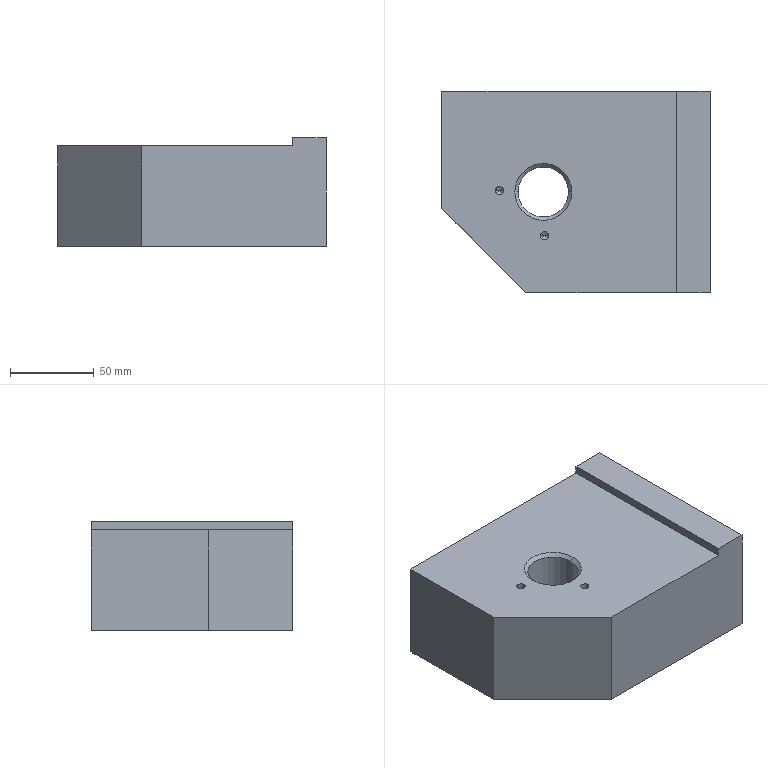Component | SolidWorks | JF21-80.1-1-3(_)-1-SOLID57-1 | 1 solid | 23 faces | box 160 x 120 x 65 mm | volume 1045468 mm3 | plane 9 | cone 8 | cylinder 6 | commonest cylinder face diameters 5 x4 30 x2
STEP:
#1=CARTESIAN_POINT('',(11.241,-3.767,39.961));
#2=VERTEX_POINT('',#1);
#3=CARTESIAN_POINT('',(12.422,-3.767,39.961));
#4=VERTEX_POINT('',#3);
#5=CARTESIAN_POINT('',(11.832,-3.767,39.961));
#6=DIRECTION('',(0.,0.,1.));
#7=DIRECTION('',(1.,0.,0.));
#8=AXIS2_PLACEMENT_3D('',#5,#6,#7);
#9=CIRCLE('',#8,0.5906);
#10=EDGE_CURVE('',#2,#4,#9,.T.);
#11=ORIENTED_EDGE('',*,*,#10,.F.);
#12=CARTESIAN_POINT('',(11.162,-3.767,40.039));
#13=VERTEX_POINT('',#12);
#14=CARTESIAN_POINT('',(11.241,-3.767,39.961));
#15=DIRECTION('',(-0.7071,0.,0.7071));
#16=VECTOR('',#15,39.37);
#17=LINE('',#14,#16);
#18=EDGE_CURVE('',#2,#13,#17,.T.);
#19=ORIENTED_EDGE('',*,*,#18,.T.);
#20=CARTESIAN_POINT('',(12.501,-3.767,40.039));
#21=VERTEX_POINT('',#20);
#22=CARTESIAN_POINT('',(11.832,-3.767,40.039));
#23=DIRECTION('',(0.,0.,-1.));
#24=DIRECTION('',(1.,0.,0.));
#25=AXIS2_PLACEMENT_3D('',#22,#23,#24);
#26=CIRCLE('',#25,0.6693);
#27=EDGE_CURVE('',#21,#13,#26,.T.);
#28=ORIENTED_EDGE('',*,*,#27,.F.);
#29=CARTESIAN_POINT('',(12.422,-3.767,39.961));
#30=DIRECTION('',(0.7071,0.,0.7071));
#31=VECTOR('',#30,39.37);
#32=LINE('',#29,#31);
#33=EDGE_CURVE('',#4,#21,#32,.T.);
#34=ORIENTED_EDGE('',*,*,#33,.F.);
#35=EDGE_LOOP('',(#11,#19,#28,#34));
#36=FACE_OUTER_BOUND('',#35,.T.);
#37=CARTESIAN_POINT('',(11.832,-3.767,39.961));
#38=DIRECTION('',(0.,0.,1.));
#39=DIRECTION('',(-1.,0.,0.));
#40=AXIS2_PLACEMENT_3D('',#37,#38,#39);
#41=CONICAL_SURFACE('',#40,0.5906,0.7854);
#42=ADVANCED_FACE('',(#36),#41,.F.);
#43=CARTESIAN_POINT('',(12.422,-3.767,37.756));
#44=VERTEX_POINT('',#43);
#45=CARTESIAN_POINT('',(11.241,-3.767,37.756));
#46=VERTEX_POINT('',#45);
#47=CARTESIAN_POINT('',(11.832,-3.767,37.756));
#48=DIRECTION('',(0.,0.,-1.));
#49=DIRECTION('',(-1.,0.,0.));
#50=AXIS2_PLACEMENT_3D('',#47,#48,#49);
#51=CIRCLE('',#50,0.5906);
#52=EDGE_CURVE('',#44,#46,#51,.T.);
#53=ORIENTED_EDGE('',*,*,#52,.F.);
#54=CARTESIAN_POINT('',(12.501,-3.767,37.677));
#55=VERTEX_POINT('',#54);
#56=CARTESIAN_POINT('',(12.501,-3.767,37.677));
#57=DIRECTION('',(-0.7071,-0.,0.7071));
#58=VECTOR('',#57,39.37);
#59=LINE('',#56,#58);
#60=EDGE_CURVE('',#55,#44,#59,.T.);
#61=ORIENTED_EDGE('',*,*,#60,.F.);
#62=CARTESIAN_POINT('',(11.162,-3.767,37.677));
#63=VERTEX_POINT('',#62);
#64=CARTESIAN_POINT('',(11.832,-3.767,37.677));
#65=DIRECTION('',(0.,0.,1.));
#66=DIRECTION('',(-1.,0.,0.));
#67=AXIS2_PLACEMENT_3D('',#64,#65,#66);
#68=CIRCLE('',#67,0.6693);
#69=EDGE_CURVE('',#63,#55,#68,.T.);
#70=ORIENTED_EDGE('',*,*,#69,.F.);
#71=CARTESIAN_POINT('',(11.162,-3.767,37.677));
#72=DIRECTION('',(0.7071,0.,0.7071));
#73=VECTOR('',#72,39.37);
#74=LINE('',#71,#73);
#75=EDGE_CURVE('',#63,#46,#74,.T.);
#76=ORIENTED_EDGE('',*,*,#75,.T.);
#77=EDGE_LOOP('',(#53,#61,#70,#76));
#78=FACE_OUTER_BOUND('',#77,.T.);
#79=CARTESIAN_POINT('',(11.832,-3.767,37.677));
#80=DIRECTION('',(0.,0.,-1.));
#81=DIRECTION('',(1.,0.,0.));
#82=AXIS2_PLACEMENT_3D('',#79,#80,#81);
#83=CONICAL_SURFACE('',#82,0.6693,0.7854);
#84=ADVANCED_FACE('',(#78),#83,.F.);
#85=CARTESIAN_POINT('',(10.703,-3.739,39.331));
#86=VERTEX_POINT('',#85);
#87=CARTESIAN_POINT('',(10.9,-3.739,39.331));
#88=VERTEX_POINT('',#87);
#89=CARTESIAN_POINT('',(10.801,-3.739,39.331));
#90=DIRECTION('',(0.,0.,1.));
#91=DIRECTION('',(1.,0.,0.));
#92=AXIS2_PLACEMENT_3D('',#89,#90,#91);
#93=CIRCLE('',#92,0.09843);
#94=EDGE_CURVE('',#86,#88,#93,.T.);
#95=ORIENTED_EDGE('',*,*,#94,.F.);
#96=CARTESIAN_POINT('',(10.703,-3.739,40.039));
#97=VERTEX_POINT('',#96);
#98=CARTESIAN_POINT('',(10.703,-3.739,40.039));
#99=DIRECTION('',(0.,0.,1.));
#100=VECTOR('',#99,39.37);
#101=LINE('',#98,#100);
#102=EDGE_CURVE('',#86,#97,#101,.T.);
#103=ORIENTED_EDGE('',*,*,#102,.T.);
#104=CARTESIAN_POINT('',(10.9,-3.739,40.039));
#105=VERTEX_POINT('',#104);
#106=CARTESIAN_POINT('',(10.801,-3.739,40.039));
#107=DIRECTION('',(0.,0.,1.));
#108=DIRECTION('',(1.,0.,0.));
#109=AXIS2_PLACEMENT_3D('',#106,#107,#108);
#110=CIRCLE('',#109,0.09843);
#111=EDGE_CURVE('',#97,#105,#110,.T.);
#112=ORIENTED_EDGE('',*,*,#111,.T.);
#113=CARTESIAN_POINT('',(10.9,-3.739,40.039));
#114=DIRECTION('',(0.,0.,1.));
#115=VECTOR('',#114,39.37);
#116=LINE('',#113,#115);
#117=EDGE_CURVE('',#88,#105,#116,.T.);
#118=ORIENTED_EDGE('',*,*,#117,.F.);
#119=EDGE_LOOP('',(#95,#103,#112,#118));
#120=FACE_OUTER_BOUND('',#119,.T.);
#121=CARTESIAN_POINT('',(10.801,-3.739,40.039));
#122=DIRECTION('',(0.,0.,1.));
#123=DIRECTION('',(-1.,0.,0.));
#124=AXIS2_PLACEMENT_3D('',#121,#122,#123);
#125=CYLINDRICAL_SURFACE('',#124,0.09843);
#126=ADVANCED_FACE('',(#120),#125,.F.);
#127=CARTESIAN_POINT('',(10.801,-3.739,39.272));
#128=VERTEX_POINT('',#127);
#129=CARTESIAN_POINT('',(10.9,-3.739,39.331));
#130=DIRECTION('',(0.8572,0.,0.515));
#131=VECTOR('',#130,39.37);
#132=LINE('',#129,#131);
#133=EDGE_CURVE('',#128,#88,#132,.T.);
#134=ORIENTED_EDGE('',*,*,#133,.F.);
#135=CARTESIAN_POINT('',(10.703,-3.739,39.331));
#136=DIRECTION('',(-0.8572,0.,0.515));
#137=VECTOR('',#136,39.37);
#138=LINE('',#135,#137);
#139=EDGE_CURVE('',#128,#86,#138,.T.);
#140=ORIENTED_EDGE('',*,*,#139,.T.);
#141=ORIENTED_EDGE('',*,*,#94,.T.);
#142=EDGE_LOOP('',(#134,#140,#141));
#143=FACE_OUTER_BOUND('',#142,.T.);
#144=CARTESIAN_POINT('',(10.801,-3.739,39.331));
#145=DIRECTION('',(0.,0.,1.));
#146=DIRECTION('',(-1.,0.,0.));
#147=AXIS2_PLACEMENT_3D('',#144,#145,#146);
#148=CONICAL_SURFACE('',#147,0.09843,1.03);
#149=ADVANCED_FACE('',(#143),#148,.F.);
#150=CARTESIAN_POINT('',(11.761,-4.797,39.331));
#151=VERTEX_POINT('',#150);
#152=CARTESIAN_POINT('',(11.958,-4.797,39.331));
#153=VERTEX_POINT('',#152);
#154=CARTESIAN_POINT('',(11.859,-4.797,39.331));
#155=DIRECTION('',(0.,0.,1.));
#156=DIRECTION('',(1.,0.,0.));
#157=AXIS2_PLACEMENT_3D('',#154,#155,#156);
#158=CIRCLE('',#157,0.09843);
#159=EDGE_CURVE('',#151,#153,#158,.T.);
#160=ORIENTED_EDGE('',*,*,#159,.F.);
#161=CARTESIAN_POINT('',(11.761,-4.797,40.039));
#162=VERTEX_POINT('',#161);
#163=CARTESIAN_POINT('',(11.761,-4.797,40.039));
#164=DIRECTION('',(0.,0.,1.));
#165=VECTOR('',#164,39.37);
#166=LINE('',#163,#165);
#167=EDGE_CURVE('',#151,#162,#166,.T.);
#168=ORIENTED_EDGE('',*,*,#167,.T.);
#169=CARTESIAN_POINT('',(11.958,-4.797,40.039));
#170=VERTEX_POINT('',#169);
#171=CARTESIAN_POINT('',(11.859,-4.797,40.039));
#172=DIRECTION('',(0.,0.,1.));
#173=DIRECTION('',(1.,0.,0.));
#174=AXIS2_PLACEMENT_3D('',#171,#172,#173);
#175=CIRCLE('',#174,0.09843);
#176=EDGE_CURVE('',#162,#170,#175,.T.);
#177=ORIENTED_EDGE('',*,*,#176,.T.);
#178=CARTESIAN_POINT('',(11.958,-4.797,40.039));
#179=DIRECTION('',(0.,0.,1.));
#180=VECTOR('',#179,39.37);
#181=LINE('',#178,#180);
#182=EDGE_CURVE('',#153,#170,#181,.T.);
#183=ORIENTED_EDGE('',*,*,#182,.F.);
#184=EDGE_LOOP('',(#160,#168,#177,#183));
#185=FACE_OUTER_BOUND('',#184,.T.);
#186=CARTESIAN_POINT('',(11.859,-4.797,40.039));
#187=DIRECTION('',(0.,0.,1.));
#188=DIRECTION('',(-1.,0.,0.));
#189=AXIS2_PLACEMENT_3D('',#186,#187,#188);
#190=CYLINDRICAL_SURFACE('',#189,0.09843);
#191=ADVANCED_FACE('',(#185),#190,.F.);
#192=CARTESIAN_POINT('',(11.859,-4.797,39.272));
#193=VERTEX_POINT('',#192);
#194=CARTESIAN_POINT('',(11.958,-4.797,39.331));
#195=DIRECTION('',(0.8572,0.,0.515));
#196=VECTOR('',#195,39.37);
#197=LINE('',#194,#196);
#198=EDGE_CURVE('',#193,#153,#197,.T.);
#199=ORIENTED_EDGE('',*,*,#198,.F.);
#200=CARTESIAN_POINT('',(11.761,-4.797,39.331));
#201=DIRECTION('',(-0.8572,0.,0.515));
#202=VECTOR('',#201,39.37);
#203=LINE('',#200,#202);
#204=EDGE_CURVE('',#193,#151,#203,.T.);
#205=ORIENTED_EDGE('',*,*,#204,.T.);
#206=ORIENTED_EDGE('',*,*,#159,.T.);
#207=EDGE_LOOP('',(#199,#205,#206));
#208=FACE_OUTER_BOUND('',#207,.T.);
#209=CARTESIAN_POINT('',(11.859,-4.797,39.331));
#210=DIRECTION('',(0.,0.,1.));
#211=DIRECTION('',(-1.,0.,0.));
#212=AXIS2_PLACEMENT_3D('',#209,#210,#211);
#213=CONICAL_SURFACE('',#212,0.09843,1.03);
#214=ADVANCED_FACE('',(#208),#213,.F.);
#215=ORIENTED_EDGE('',*,*,#10,.T.);
#216=CARTESIAN_POINT('',(12.422,-3.767,40.236));
#217=DIRECTION('',(0.,0.,1.));
#218=VECTOR('',#217,39.37);
#219=LINE('',#216,#218);
#220=EDGE_CURVE('',#44,#4,#219,.T.);
#221=ORIENTED_EDGE('',*,*,#220,.F.);
#222=ORIENTED_EDGE('',*,*,#52,.T.);
#223=CARTESIAN_POINT('',(11.241,-3.767,40.236));
#224=DIRECTION('',(0.,0.,1.));
#225=VECTOR('',#224,39.37);
#226=LINE('',#223,#225);
#227=EDGE_CURVE('',#46,#2,#226,.T.);
#228=ORIENTED_EDGE('',*,*,#227,.T.);
#229=EDGE_LOOP('',(#215,#221,#222,#228));
#230=FACE_OUTER_BOUND('',#229,.T.);
#231=CARTESIAN_POINT('',(11.832,-3.767,40.236));
#232=DIRECTION('',(0.,0.,-1.));
#233=DIRECTION('',(1.,0.,0.));
#234=AXIS2_PLACEMENT_3D('',#231,#232,#233);
#235=CYLINDRICAL_SURFACE('',#234,0.5906);
#236=ADVANCED_FACE('',(#230),#235,.F.);
#237=CARTESIAN_POINT('',(9.449,-1.404,40.039));
#238=VERTEX_POINT('',#237);
#239=CARTESIAN_POINT('',(9.449,-4.16,40.039));
#240=VERTEX_POINT('',#239);
#241=CARTESIAN_POINT('',(9.449,-1.404,40.039));
#242=DIRECTION('',(0.,-1.,0.));
#243=VECTOR('',#242,39.37);
#244=LINE('',#241,#243);
#245=EDGE_CURVE('',#238,#240,#244,.T.);
#246=ORIENTED_EDGE('',*,*,#245,.F.);
#247=CARTESIAN_POINT('',(9.449,-1.404,37.677));
#248=VERTEX_POINT('',#247);
#249=CARTESIAN_POINT('',(9.449,-1.404,40.236));
#250=DIRECTION('',(0.,0.,-1.));
#251=VECTOR('',#250,39.37);
#252=LINE('',#249,#251);
#253=EDGE_CURVE('',#238,#248,#252,.T.);
#254=ORIENTED_EDGE('',*,*,#253,.T.);
#255=CARTESIAN_POINT('',(9.449,-4.16,37.677));
#256=VERTEX_POINT('',#255);
#257=CARTESIAN_POINT('',(9.449,-1.404,37.677));
#258=DIRECTION('',(0.,-1.,0.));
#259=VECTOR('',#258,39.37);
#260=LINE('',#257,#259);
#261=EDGE_CURVE('',#248,#256,#260,.T.);
#262=ORIENTED_EDGE('',*,*,#261,.T.);
#263=CARTESIAN_POINT('',(9.449,-4.16,40.236));
#264=DIRECTION('',(0.,0.,-1.));
#265=VECTOR('',#264,39.37);
#266=LINE('',#263,#265);
#267=EDGE_CURVE('',#240,#256,#266,.T.);
#268=ORIENTED_EDGE('',*,*,#267,.F.);
#269=EDGE_LOOP('',(#246,#254,#262,#268));
#270=FACE_OUTER_BOUND('',#269,.T.);
#271=CARTESIAN_POINT('',(9.449,-1.404,40.236));
#272=DIRECTION('',(1.,0.,0.));
#273=DIRECTION('',(0.,0.,1.));
#274=AXIS2_PLACEMENT_3D('',#271,#272,#273);
#275=PLANE('',#274);
#276=ADVANCED_FACE('',(#270),#275,.F.);
#277=CARTESIAN_POINT('',(11.417,-6.129,40.039));
#278=VERTEX_POINT('',#277);
#279=CARTESIAN_POINT('',(9.449,-4.16,40.039));
#280=DIRECTION('',(0.7071,-0.7071,0.));
#281=VECTOR('',#280,39.37);
#282=LINE('',#279,#281);
#283=EDGE_CURVE('',#240,#278,#282,.T.);
#284=ORIENTED_EDGE('',*,*,#283,.F.);
#285=ORIENTED_EDGE('',*,*,#267,.T.);
#286=CARTESIAN_POINT('',(11.417,-6.129,37.677));
#287=VERTEX_POINT('',#286);
#288=CARTESIAN_POINT('',(9.449,-4.16,37.677));
#289=DIRECTION('',(0.7071,-0.7071,0.));
#290=VECTOR('',#289,39.37);
#291=LINE('',#288,#290);
#292=EDGE_CURVE('',#256,#287,#291,.T.);
#293=ORIENTED_EDGE('',*,*,#292,.T.);
#294=CARTESIAN_POINT('',(11.417,-6.129,40.236));
#295=DIRECTION('',(0.,0.,-1.));
#296=VECTOR('',#295,39.37);
#297=LINE('',#294,#296);
#298=EDGE_CURVE('',#278,#287,#297,.T.);
#299=ORIENTED_EDGE('',*,*,#298,.F.);
#300=EDGE_LOOP('',(#284,#285,#293,#299));
#301=FACE_OUTER_BOUND('',#300,.T.);
#302=CARTESIAN_POINT('',(9.449,-4.16,40.236));
#303=DIRECTION('',(0.7071,0.7071,0.));
#304=DIRECTION('',(0.7071,-0.7071,0.));
#305=AXIS2_PLACEMENT_3D('',#302,#303,#304);
#306=PLANE('',#305);
#307=ADVANCED_FACE('',(#301),#306,.F.);
#308=ORIENTED_EDGE('',*,*,#220,.T.);
#309=CARTESIAN_POINT('',(11.832,-3.767,39.961));
#310=DIRECTION('',(0.,0.,1.));
#311=DIRECTION('',(1.,0.,0.));
#312=AXIS2_PLACEMENT_3D('',#309,#310,#311);
#313=CIRCLE('',#312,0.5906);
#314=EDGE_CURVE('',#4,#2,#313,.T.);
#315=ORIENTED_EDGE('',*,*,#314,.T.);
#316=ORIENTED_EDGE('',*,*,#227,.F.);
#317=CARTESIAN_POINT('',(11.832,-3.767,37.756));
#318=DIRECTION('',(0.,0.,-1.));
#319=DIRECTION('',(-1.,0.,0.));
#320=AXIS2_PLACEMENT_3D('',#317,#318,#319);
#321=CIRCLE('',#320,0.5906);
#322=EDGE_CURVE('',#46,#44,#321,.T.);
#323=ORIENTED_EDGE('',*,*,#322,.T.);
#324=EDGE_LOOP('',(#308,#315,#316,#323));
#325=FACE_OUTER_BOUND('',#324,.T.);
#326=CARTESIAN_POINT('',(11.832,-3.767,40.236));
#327=DIRECTION('',(0.,0.,-1.));
#328=DIRECTION('',(1.,0.,0.));
#329=AXIS2_PLACEMENT_3D('',#326,#327,#328);
#330=CYLINDRICAL_SURFACE('',#329,0.5906);
#331=ADVANCED_FACE('',(#325),#330,.F.);
#332=CARTESIAN_POINT('',(15.748,-1.404,40.236));
#333=VERTEX_POINT('',#332);
#334=CARTESIAN_POINT('',(14.961,-1.404,40.236));
#335=VERTEX_POINT('',#334);
#336=CARTESIAN_POINT('',(15.748,-1.404,40.236));
#337=DIRECTION('',(-1.,-0.,0.));
#338=VECTOR('',#337,39.37);
#339=LINE('',#336,#338);
#340=EDGE_CURVE('',#333,#335,#339,.T.);
#341=ORIENTED_EDGE('',*,*,#340,.T.);
#342=CARTESIAN_POINT('',(14.961,-6.129,40.236));
#343=VERTEX_POINT('',#342);
#344=CARTESIAN_POINT('',(14.961,-1.404,40.236));
#345=DIRECTION('',(0.,1.,0.));
#346=VECTOR('',#345,39.37);
#347=LINE('',#344,#346);
#348=EDGE_CURVE('',#343,#335,#347,.T.);
#349=ORIENTED_EDGE('',*,*,#348,.F.);
#350=CARTESIAN_POINT('',(15.748,-6.129,40.236));
#351=VERTEX_POINT('',#350);
#352=CARTESIAN_POINT('',(15.748,-6.129,40.236));
#353=DIRECTION('',(1.,0.,0.));
#354=VECTOR('',#353,39.37);
#355=LINE('',#352,#354);
#356=EDGE_CURVE('',#343,#351,#355,.T.);
#357=ORIENTED_EDGE('',*,*,#356,.T.);
#358=CARTESIAN_POINT('',(15.748,-1.404,40.236));
#359=DIRECTION('',(0.,1.,0.));
#360=VECTOR('',#359,39.37);
#361=LINE('',#358,#360);
#362=EDGE_CURVE('',#351,#333,#361,.T.);
#363=ORIENTED_EDGE('',*,*,#362,.T.);
#364=EDGE_LOOP('',(#341,#349,#357,#363));
#365=FACE_OUTER_BOUND('',#364,.T.);
#366=CARTESIAN_POINT('',(15.748,-6.129,40.236));
#367=DIRECTION('',(0.,0.,-1.));
#368=DIRECTION('',(1.,0.,0.));
#369=AXIS2_PLACEMENT_3D('',#366,#367,#368);
#370=PLANE('',#369);
#371=ADVANCED_FACE('',(#365),#370,.F.);
#372=ORIENTED_EDGE('',*,*,#69,.T.);
#373=CARTESIAN_POINT('',(11.832,-3.767,37.677));
#374=DIRECTION('',(0.,0.,1.));
#375=DIRECTION('',(-1.,0.,0.));
#376=AXIS2_PLACEMENT_3D('',#373,#374,#375);
#377=CIRCLE('',#376,0.6693);
#378=EDGE_CURVE('',#55,#63,#377,.T.);
#379=ORIENTED_EDGE('',*,*,#378,.T.);
#380=EDGE_LOOP('',(#372,#379));
#381=FACE_BOUND('',#380,.T.);
#382=CARTESIAN_POINT('',(15.748,-6.129,37.677));
#383=VERTEX_POINT('',#382);
#384=CARTESIAN_POINT('',(15.748,-1.404,37.677));
#385=VERTEX_POINT('',#384);
#386=CARTESIAN_POINT('',(15.748,-1.404,37.677));
#387=DIRECTION('',(0.,1.,0.));
#388=VECTOR('',#387,39.37);
#389=LINE('',#386,#388);
#390=EDGE_CURVE('',#383,#385,#389,.T.);
#391=ORIENTED_EDGE('',*,*,#390,.F.);
#392=CARTESIAN_POINT('',(15.748,-6.129,37.677));
#393=DIRECTION('',(1.,0.,0.));
#394=VECTOR('',#393,39.37);
#395=LINE('',#392,#394);
#396=EDGE_CURVE('',#287,#383,#395,.T.);
#397=ORIENTED_EDGE('',*,*,#396,.F.);
#398=ORIENTED_EDGE('',*,*,#292,.F.);
#399=ORIENTED_EDGE('',*,*,#261,.F.);
#400=CARTESIAN_POINT('',(15.748,-1.404,37.677));
#401=DIRECTION('',(-1.,-0.,0.));
#402=VECTOR('',#401,39.37);
#403=LINE('',#400,#402);
#404=EDGE_CURVE('',#385,#248,#403,.T.);
#405=ORIENTED_EDGE('',*,*,#404,.F.);
#406=EDGE_LOOP('',(#391,#397,#398,#399,#405));
#407=FACE_OUTER_BOUND('',#406,.T.);
#408=CARTESIAN_POINT('',(15.748,-6.129,37.677));
#409=DIRECTION('',(0.,0.,-1.));
#410=DIRECTION('',(1.,0.,0.));
#411=AXIS2_PLACEMENT_3D('',#408,#409,#410);
#412=PLANE('',#411);
#413=ADVANCED_FACE('',(#381,#407),#412,.T.);
#414=ORIENTED_EDGE('',*,*,#390,.T.);
#415=CARTESIAN_POINT('',(15.748,-1.404,40.236));
#416=DIRECTION('',(0.,0.,-1.));
#417=VECTOR('',#416,39.37);
#418=LINE('',#415,#417);
#419=EDGE_CURVE('',#333,#385,#418,.T.);
#420=ORIENTED_EDGE('',*,*,#419,.F.);
#421=ORIENTED_EDGE('',*,*,#362,.F.);
#422=CARTESIAN_POINT('',(15.748,-6.129,40.236));
#423=DIRECTION('',(0.,0.,-1.));
#424=VECTOR('',#423,39.37);
#425=LINE('',#422,#424);
#426=EDGE_CURVE('',#351,#383,#425,.T.);
#427=ORIENTED_EDGE('',*,*,#426,.T.);
#428=EDGE_LOOP('',(#414,#420,#421,#427));
#429=FACE_OUTER_BOUND('',#428,.T.);
#430=CARTESIAN_POINT('',(15.748,-1.404,40.236));
#431=DIRECTION('',(-1.,0.,0.));
#432=DIRECTION('',(0.,0.,-1.));
#433=AXIS2_PLACEMENT_3D('',#430,#431,#432);
#434=PLANE('',#433);
#435=ADVANCED_FACE('',(#429),#434,.F.);
#436=CARTESIAN_POINT('',(14.961,-1.404,40.039));
#437=VERTEX_POINT('',#436);
#438=CARTESIAN_POINT('',(14.961,-1.404,40.039));
#439=DIRECTION('',(-1.,-0.,0.));
#440=VECTOR('',#439,39.37);
#441=LINE('',#438,#440);
#442=EDGE_CURVE('',#437,#238,#441,.T.);
#443=ORIENTED_EDGE('',*,*,#442,.F.);
#444=CARTESIAN_POINT('',(14.961,-1.404,40.039));
#445=DIRECTION('',(0.,0.,1.));
#446=VECTOR('',#445,39.37);
#447=LINE('',#444,#446);
#448=EDGE_CURVE('',#437,#335,#447,.T.);
#449=ORIENTED_EDGE('',*,*,#448,.T.);
#450=ORIENTED_EDGE('',*,*,#340,.F.);
#451=ORIENTED_EDGE('',*,*,#419,.T.);
#452=ORIENTED_EDGE('',*,*,#404,.T.);
#453=ORIENTED_EDGE('',*,*,#253,.F.);
#454=EDGE_LOOP('',(#443,#449,#450,#451,#452,#453));
#455=FACE_OUTER_BOUND('',#454,.T.);
#456=CARTESIAN_POINT('',(15.748,-1.404,40.236));
#457=DIRECTION('',(0.,-1.,0.));
#458=DIRECTION('',(-1.,-0.,0.));
#459=AXIS2_PLACEMENT_3D('',#456,#457,#458);
#460=PLANE('',#459);
#461=ADVANCED_FACE('',(#455),#460,.F.);
#462=ORIENTED_EDGE('',*,*,#356,.F.);
#463=CARTESIAN_POINT('',(14.961,-6.129,40.039));
#464=VERTEX_POINT('',#463);
#465=CARTESIAN_POINT('',(14.961,-6.129,40.039));
#466=DIRECTION('',(0.,0.,1.));
#467=VECTOR('',#466,39.37);
#468=LINE('',#465,#467);
#469=EDGE_CURVE('',#464,#343,#468,.T.);
#470=ORIENTED_EDGE('',*,*,#469,.F.);
#471=CARTESIAN_POINT('',(11.417,-6.129,40.039));
#472=DIRECTION('',(1.,0.,0.));
#473=VECTOR('',#472,39.37);
#474=LINE('',#471,#473);
#475=EDGE_CURVE('',#278,#464,#474,.T.);
#476=ORIENTED_EDGE('',*,*,#475,.F.);
#477=ORIENTED_EDGE('',*,*,#298,.T.);
#478=ORIENTED_EDGE('',*,*,#396,.T.);
#479=ORIENTED_EDGE('',*,*,#426,.F.);
#480=EDGE_LOOP('',(#462,#470,#476,#477,#478,#479));
#481=FACE_OUTER_BOUND('',#480,.T.);
#482=CARTESIAN_POINT('',(15.748,-6.129,40.236));
#483=DIRECTION('',(0.,1.,0.));
#484=DIRECTION('',(0.,0.,-1.));
#485=AXIS2_PLACEMENT_3D('',#482,#483,#484);
#486=PLANE('',#485);
#487=ADVANCED_FACE('',(#481),#486,.F.);
#488=ORIENTED_EDGE('',*,*,#348,.T.);
#489=ORIENTED_EDGE('',*,*,#448,.F.);
#490=CARTESIAN_POINT('',(14.961,-1.404,40.039));
#491=DIRECTION('',(0.,1.,0.));
#492=VECTOR('',#491,39.37);
#493=LINE('',#490,#492);
#494=EDGE_CURVE('',#464,#437,#493,.T.);
#495=ORIENTED_EDGE('',*,*,#494,.F.);
#496=ORIENTED_EDGE('',*,*,#469,.T.);
#497=EDGE_LOOP('',(#488,#489,#495,#496));
#498=FACE_OUTER_BOUND('',#497,.T.);
#499=CARTESIAN_POINT('',(14.961,-1.404,40.039));
#500=DIRECTION('',(1.,0.,0.));
#501=DIRECTION('',(0.,0.,1.));
#502=AXIS2_PLACEMENT_3D('',#499,#500,#501);
#503=PLANE('',#502);
#504=ADVANCED_FACE('',(#498),#503,.F.);
#505=ORIENTED_EDGE('',*,*,#27,.T.);
#506=CARTESIAN_POINT('',(11.832,-3.767,40.039));
#507=DIRECTION('',(0.,0.,-1.));
#508=DIRECTION('',(1.,0.,0.));
#509=AXIS2_PLACEMENT_3D('',#506,#507,#508);
#510=CIRCLE('',#509,0.6693);
#511=EDGE_CURVE('',#13,#21,#510,.T.);
#512=ORIENTED_EDGE('',*,*,#511,.T.);
#513=EDGE_LOOP('',(#505,#512));
#514=FACE_BOUND('',#513,.T.);
#515=CARTESIAN_POINT('',(10.801,-3.739,40.039));
#516=DIRECTION('',(0.,0.,1.));
#517=DIRECTION('',(1.,0.,0.));
#518=AXIS2_PLACEMENT_3D('',#515,#516,#517);
#519=CIRCLE('',#518,0.09843);
#520=EDGE_CURVE('',#105,#97,#519,.T.);
#521=ORIENTED_EDGE('',*,*,#520,.F.);
#522=ORIENTED_EDGE('',*,*,#111,.F.);
#523=EDGE_LOOP('',(#521,#522));
#524=FACE_BOUND('',#523,.T.);
#525=CARTESIAN_POINT('',(11.859,-4.797,40.039));
#526=DIRECTION('',(0.,0.,1.));
#527=DIRECTION('',(1.,0.,0.));
#528=AXIS2_PLACEMENT_3D('',#525,#526,#527);
#529=CIRCLE('',#528,0.09843);
#530=EDGE_CURVE('',#170,#162,#529,.T.);
#531=ORIENTED_EDGE('',*,*,#530,.F.);
#532=ORIENTED_EDGE('',*,*,#176,.F.);
#533=EDGE_LOOP('',(#531,#532));
#534=FACE_BOUND('',#533,.T.);
#535=ORIENTED_EDGE('',*,*,#283,.T.);
#536=ORIENTED_EDGE('',*,*,#475,.T.);
#537=ORIENTED_EDGE('',*,*,#494,.T.);
#538=ORIENTED_EDGE('',*,*,#442,.T.);
#539=ORIENTED_EDGE('',*,*,#245,.T.);
#540=EDGE_LOOP('',(#535,#536,#537,#538,#539));
#541=FACE_OUTER_BOUND('',#540,.T.);
#542=CARTESIAN_POINT('',(11.417,-6.129,40.039));
#543=DIRECTION('',(0.,0.,1.));
#544=DIRECTION('',(-1.,0.,0.));
#545=AXIS2_PLACEMENT_3D('',#542,#543,#544);
#546=PLANE('',#545);
#547=ADVANCED_FACE('',(#514,#524,#534,#541),#546,.T.);
#548=ORIENTED_EDGE('',*,*,#204,.F.);
#549=ORIENTED_EDGE('',*,*,#198,.T.);
#550=CARTESIAN_POINT('',(11.859,-4.797,39.331));
#551=DIRECTION('',(0.,0.,1.));
#552=DIRECTION('',(1.,0.,0.));
#553=AXIS2_PLACEMENT_3D('',#550,#551,#552);
#554=CIRCLE('',#553,0.09843);
#555=EDGE_CURVE('',#153,#151,#554,.T.);
#556=ORIENTED_EDGE('',*,*,#555,.T.);
#557=EDGE_LOOP('',(#548,#549,#556));
#558=FACE_OUTER_BOUND('',#557,.T.);
#559=CARTESIAN_POINT('',(11.859,-4.797,39.331));
#560=DIRECTION('',(0.,0.,1.));
#561=DIRECTION('',(-1.,0.,0.));
#562=AXIS2_PLACEMENT_3D('',#559,#560,#561);
#563=CONICAL_SURFACE('',#562,0.09843,1.03);
#564=ADVANCED_FACE('',(#558),#563,.F.);
#565=ORIENTED_EDGE('',*,*,#167,.F.);
#566=ORIENTED_EDGE('',*,*,#555,.F.);
#567=ORIENTED_EDGE('',*,*,#182,.T.);
#568=ORIENTED_EDGE('',*,*,#530,.T.);
#569=EDGE_LOOP('',(#565,#566,#567,#568));
#570=FACE_OUTER_BOUND('',#569,.T.);
#571=CARTESIAN_POINT('',(11.859,-4.797,40.039));
#572=DIRECTION('',(0.,0.,1.));
#573=DIRECTION('',(-1.,0.,0.));
#574=AXIS2_PLACEMENT_3D('',#571,#572,#573);
#575=CYLINDRICAL_SURFACE('',#574,0.09843);
#576=ADVANCED_FACE('',(#570),#575,.F.);
#577=ORIENTED_EDGE('',*,*,#139,.F.);
#578=ORIENTED_EDGE('',*,*,#133,.T.);
#579=CARTESIAN_POINT('',(10.801,-3.739,39.331));
#580=DIRECTION('',(0.,0.,1.));
#581=DIRECTION('',(1.,0.,0.));
#582=AXIS2_PLACEMENT_3D('',#579,#580,#581);
#583=CIRCLE('',#582,0.09843);
#584=EDGE_CURVE('',#88,#86,#583,.T.);
#585=ORIENTED_EDGE('',*,*,#584,.T.);
#586=EDGE_LOOP('',(#577,#578,#585));
#587=FACE_OUTER_BOUND('',#586,.T.);
#588=CARTESIAN_POINT('',(10.801,-3.739,39.331));
#589=DIRECTION('',(0.,0.,1.));
#590=DIRECTION('',(-1.,0.,0.));
#591=AXIS2_PLACEMENT_3D('',#588,#589,#590);
#592=CONICAL_SURFACE('',#591,0.09843,1.03);
#593=ADVANCED_FACE('',(#587),#592,.F.);
#594=ORIENTED_EDGE('',*,*,#102,.F.);
#595=ORIENTED_EDGE('',*,*,#584,.F.);
#596=ORIENTED_EDGE('',*,*,#117,.T.);
#597=ORIENTED_EDGE('',*,*,#520,.T.);
#598=EDGE_LOOP('',(#594,#595,#596,#597));
#599=FACE_OUTER_BOUND('',#598,.T.);
#600=CARTESIAN_POINT('',(10.801,-3.739,40.039));
#601=DIRECTION('',(0.,0.,1.));
#602=DIRECTION('',(-1.,0.,0.));
#603=AXIS2_PLACEMENT_3D('',#600,#601,#602);
#604=CYLINDRICAL_SURFACE('',#603,0.09843);
#605=ADVANCED_FACE('',(#599),#604,.F.);
#606=ORIENTED_EDGE('',*,*,#60,.T.);
#607=ORIENTED_EDGE('',*,*,#322,.F.);
#608=ORIENTED_EDGE('',*,*,#75,.F.);
#609=ORIENTED_EDGE('',*,*,#378,.F.);
#610=EDGE_LOOP('',(#606,#607,#608,#609));
#611=FACE_OUTER_BOUND('',#610,.T.);
#612=CARTESIAN_POINT('',(11.832,-3.767,37.677));
#613=DIRECTION('',(0.,0.,-1.));
#614=DIRECTION('',(1.,0.,0.));
#615=AXIS2_PLACEMENT_3D('',#612,#613,#614);
#616=CONICAL_SURFACE('',#615,0.6693,0.7854);
#617=ADVANCED_FACE('',(#611),#616,.F.);
#618=ORIENTED_EDGE('',*,*,#18,.F.);
#619=ORIENTED_EDGE('',*,*,#314,.F.);
#620=ORIENTED_EDGE('',*,*,#33,.T.);
#621=ORIENTED_EDGE('',*,*,#511,.F.);
#622=EDGE_LOOP('',(#618,#619,#620,#621));
#623=FACE_OUTER_BOUND('',#622,.T.);
#624=CARTESIAN_POINT('',(11.832,-3.767,39.961));
#625=DIRECTION('',(0.,0.,1.));
#626=DIRECTION('',(-1.,0.,0.));
#627=AXIS2_PLACEMENT_3D('',#624,#625,#626);
#628=CONICAL_SURFACE('',#627,0.5906,0.7854);
#629=ADVANCED_FACE('',(#623),#628,.F.);
#630=CLOSED_SHELL('',(#42,#84,#126,#149,#191,#214,#236,#276,#307,#331,#371,#413,#435,#461,#487,#504,#547,#564,#576,#593,#605,#617,#629));
#631=MANIFOLD_SOLID_BREP('',#630);
#632=CARTESIAN_POINT('',(0.,0.,0.));
#633=DIRECTION('',(0.,0.,1.));
#634=DIRECTION('',(1.,0.,0.));
#635=AXIS2_PLACEMENT_3D('',#632,#633,#634);
#636=(LENGTH_UNIT()NAMED_UNIT(*)SI_UNIT($,.METRE.));
#637=LENGTH_MEASURE_WITH_UNIT(LENGTH_MEASURE(0.0254),#636);
#638=DIMENSIONAL_EXPONENTS(1.,0.,0.,0.,0.,0.,0.);
#639=(CONVERSION_BASED_UNIT('',#637)LENGTH_UNIT()NAMED_UNIT(#638));
#640=UNCERTAINTY_MEASURE_WITH_UNIT(LENGTH_MEASURE(0.00001),#639,'','');
#641=(NAMED_UNIT(*)PLANE_ANGLE_UNIT()SI_UNIT($,.RADIAN.));
#642=(NAMED_UNIT(*)SI_UNIT($,.STERADIAN.)SOLID_ANGLE_UNIT());
#643=(GEOMETRIC_REPRESENTATION_CONTEXT(3)GLOBAL_UNCERTAINTY_ASSIGNED_CONTEXT((#640))GLOBAL_UNIT_ASSIGNED_CONTEXT((#639,#641,#642))REPRESENTATION_CONTEXT('',''));
#644=ADVANCED_BREP_SHAPE_REPRESENTATION('',(#631,#635),#643);
#645=COLOUR_RGB('',0.7922,0.8196,0.9333);
#646=FILL_AREA_STYLE_COLOUR('',#645);
#647=FILL_AREA_STYLE('',(#646));
#648=SURFACE_STYLE_FILL_AREA(#647);
#649=SURFACE_SIDE_STYLE('',(#648));
#650=SURFACE_STYLE_USAGE(.BOTH.,#649);
#651=PRESENTATION_STYLE_ASSIGNMENT((#650));
#652=STYLED_ITEM('',(#651),#631);
#653=PRESENTATION_LAYER_ASSIGNMENT('','',(#652));
#654=(LENGTH_UNIT()NAMED_UNIT(*)SI_UNIT($,.METRE.));
#655=LENGTH_MEASURE_WITH_UNIT(LENGTH_MEASURE(0.0254),#654);
#656=DIMENSIONAL_EXPONENTS(1.,0.,0.,0.,0.,0.,0.);
#657=(CONVERSION_BASED_UNIT('',#655)LENGTH_UNIT()NAMED_UNIT(#656));
#658=UNCERTAINTY_MEASURE_WITH_UNIT(LENGTH_MEASURE(0.00001),#657,'','');
#659=(NAMED_UNIT(*)PLANE_ANGLE_UNIT()SI_UNIT($,.RADIAN.));
#660=(NAMED_UNIT(*)SI_UNIT($,.STERADIAN.)SOLID_ANGLE_UNIT());
#661=(GEOMETRIC_REPRESENTATION_CONTEXT(3)GLOBAL_UNCERTAINTY_ASSIGNED_CONTEXT((#658))GLOBAL_UNIT_ASSIGNED_CONTEXT((#657,#659,#660))REPRESENTATION_CONTEXT('',''));
#662=MECHANICAL_DESIGN_GEOMETRIC_PRESENTATION_REPRESENTATION('',(#652),#661);